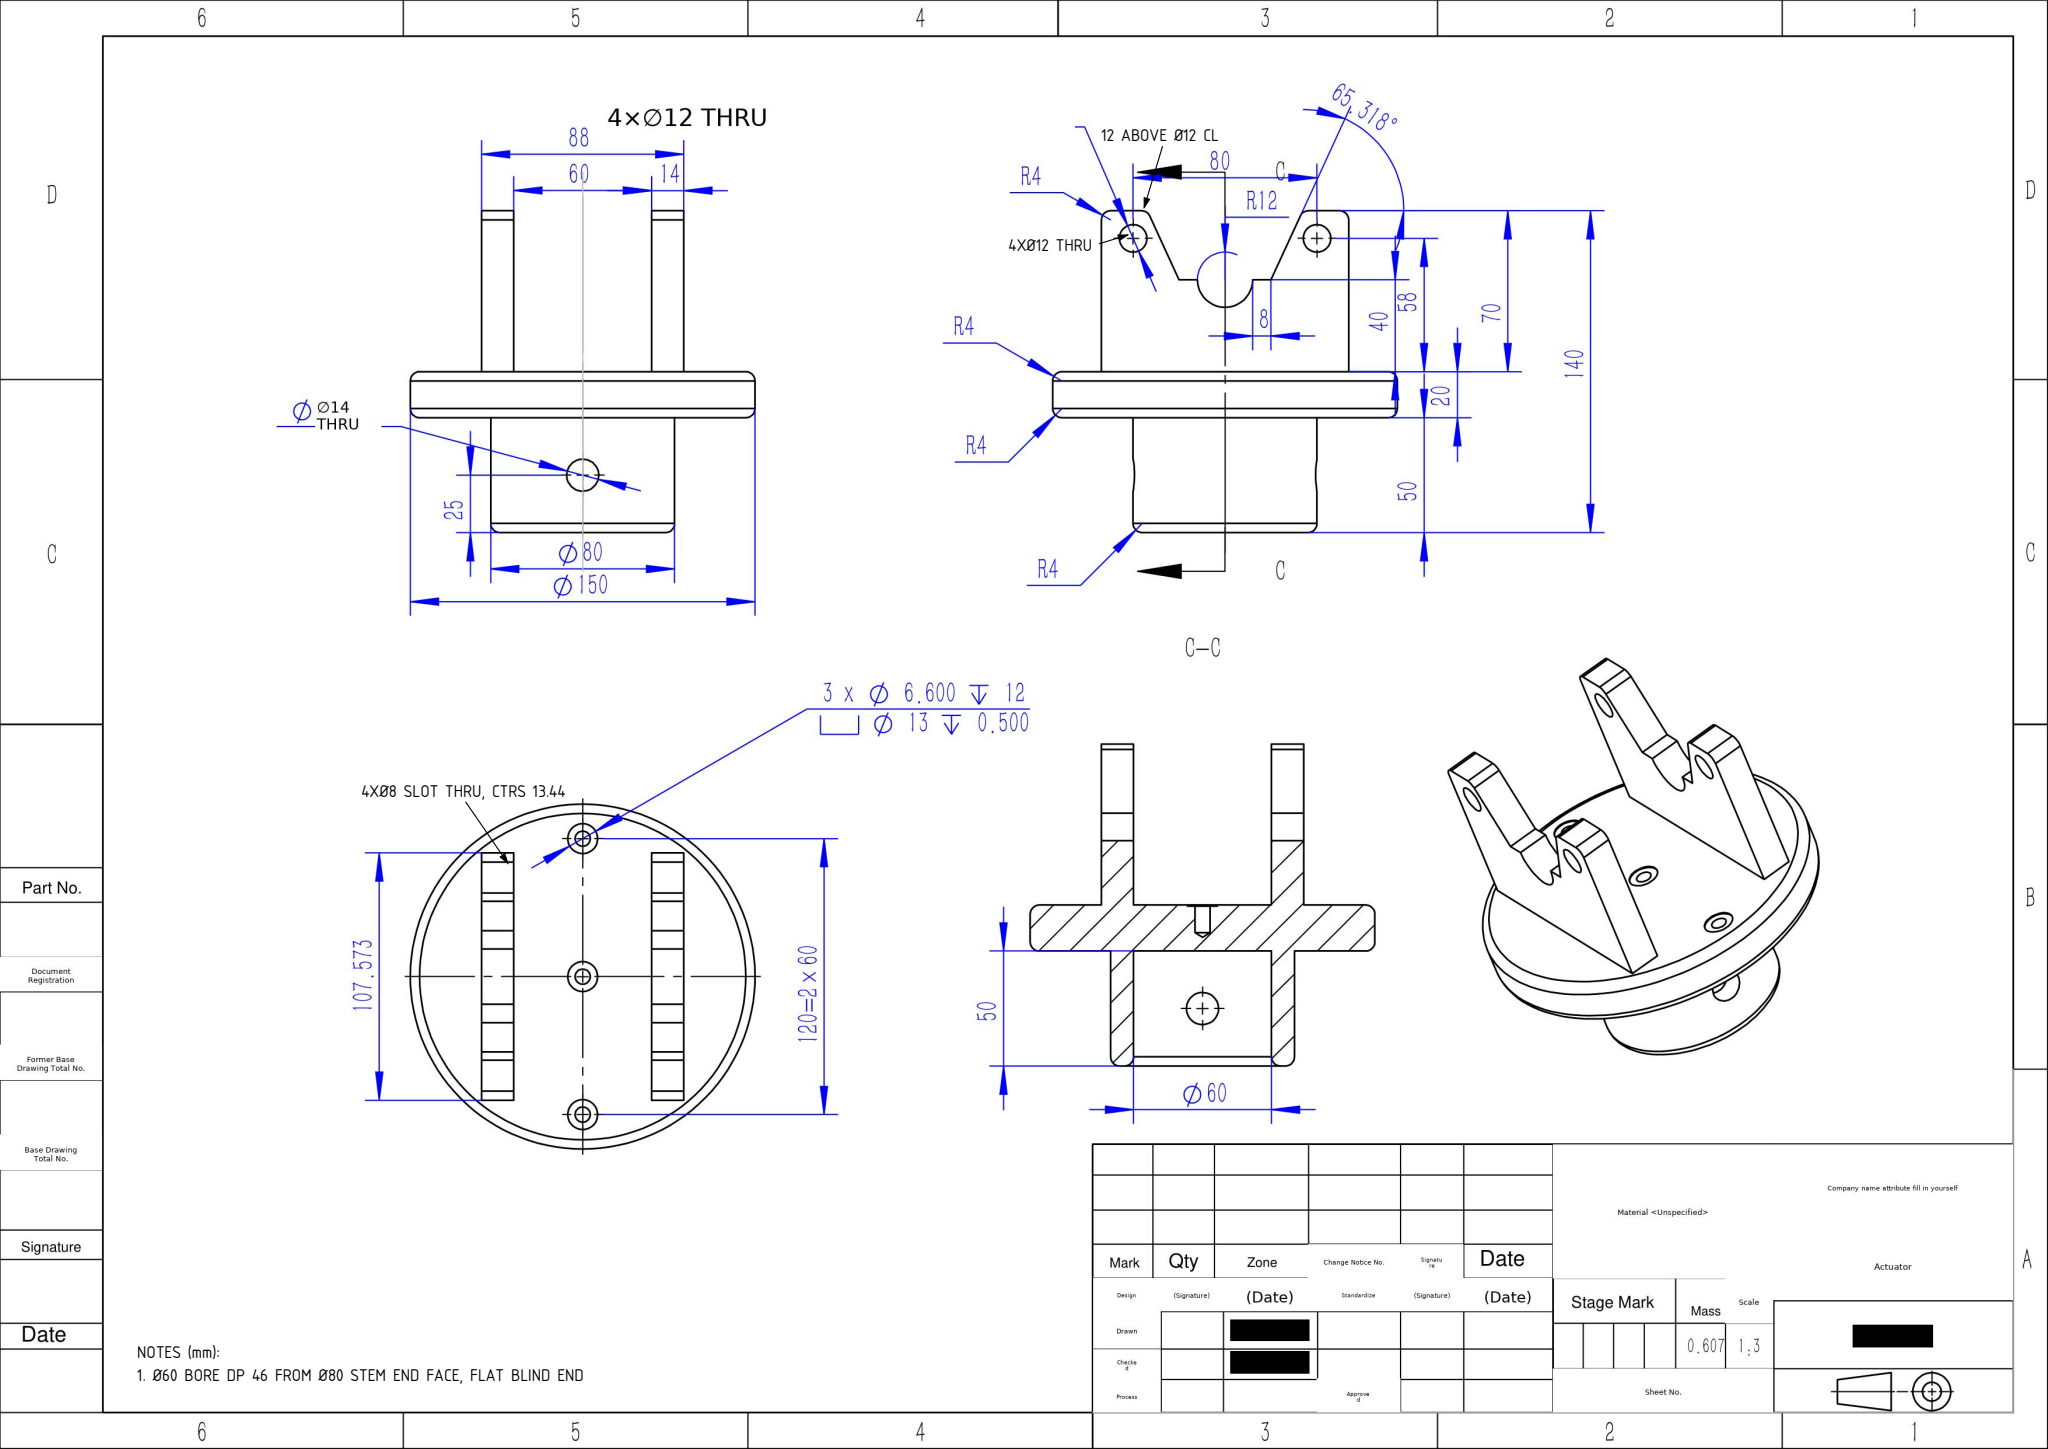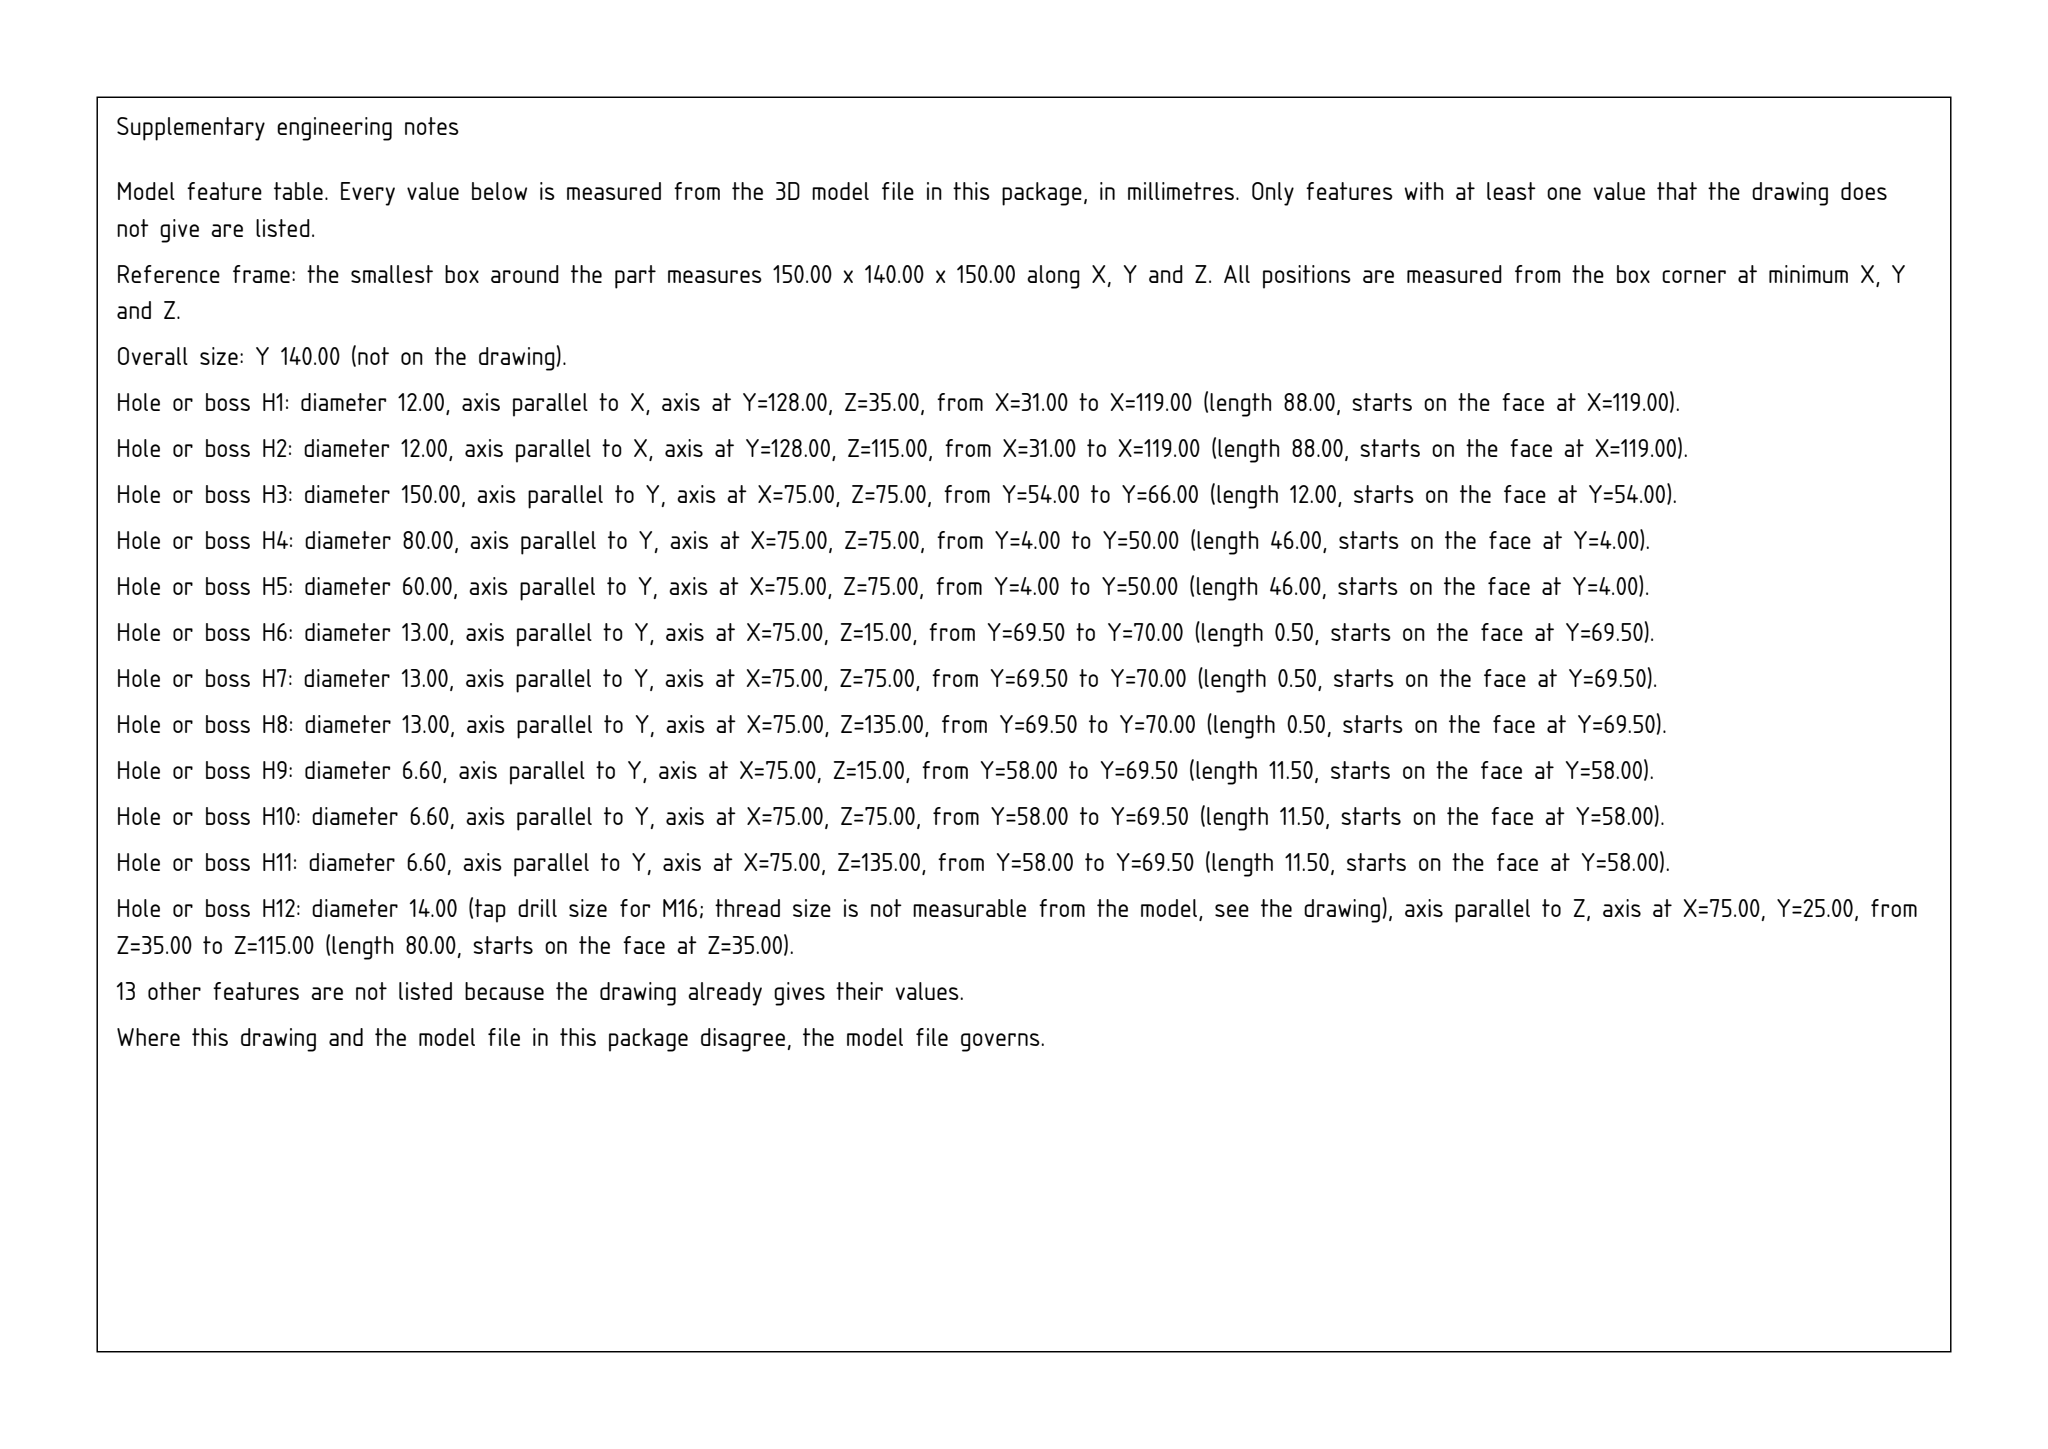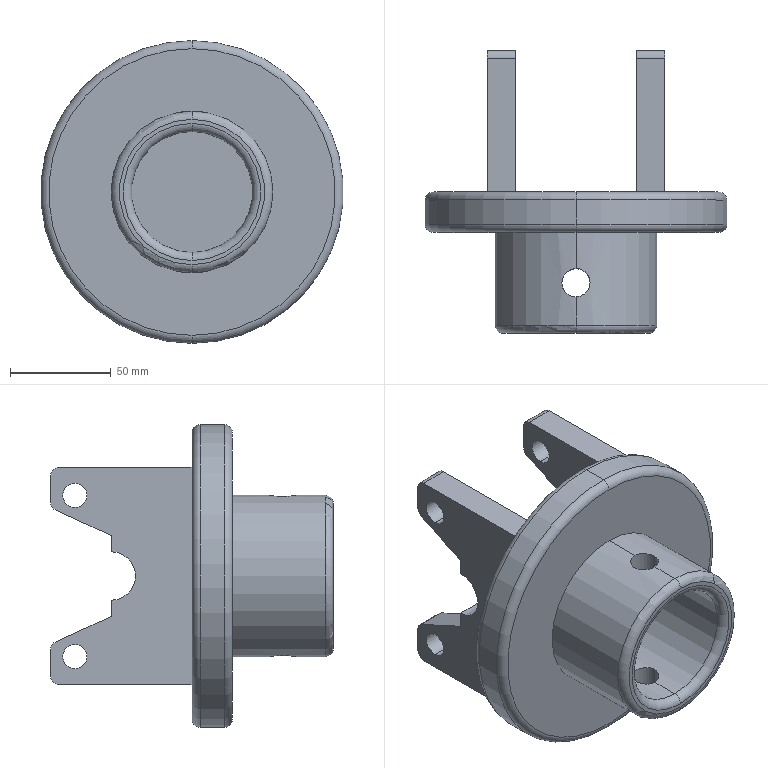Part | SolidWorks | mm | 1 solid | 81 faces | box 150 x 140 x 150 mm | volume 606876 mm3 | cylinder 40 | plane 27 | torus 8 | cone 6 | commonest cylinder face diameters 12 x8 8 x8 13 x6 6.6 x6 14 x4 150 x2 60 x2 80 x2
Drawing notes:
Ø60 BORE DP 46 FROM Ø80 STEM END FACE, FLAT BLIND END | from the solid: Ø60 y-axis cyl at [81.18,81.18] len 46; starts at stem end y=0, ends y=50, 4 below flange underside
4×Ø12 THRU AXES PERP FLANGE AXIS, 80 APART SYM ABT CL, CL 58 ABV FLANGE TOP | from the solid: Ø12 x-axis cyls at y=128, z=41.18 & 121.18; flange axis z=81.18 (±40); flange top plane y=70 → 128-70=58
PRONG TIP END FACE 12 ABV Ø12 CL; PRONG OUTR FACE 13.79 FROM Ø12 CL | from the solid: tip end face y=140 vs Ø12 axis y=128 → 12; Ø12 at z=41.18 vs prong outer face z=27.39 → 13.79
4×Ø8 THRU SLOT: CTRS 13.44 APART, 4 & 17.44 FROM PRONG OUTR FACE, CL 66 ABV FLANGE TOP | from the solid: Ø8 x-axis cyls y=136, z=31.39 & 44.83 (and 117.53 & 130.97), len 14 = prong thk; outer faces z=27.39/134.97; 136-70=66
build123d program:
from build123d import *

# Parameters (mm, degrees)
SKETCH1_R                                           = 40
SKETCH1_R_2                                         = 30
BOSS_EXTRUDE1_DEPTH                                 = 50
SKETCH2_R                                           = 75
BOSS_EXTRUDE2_DEPTH                                 = 20
BOSS_EXTRUDE3_START                                 = 30
BOSS_EXTRUDE3_DEPTH                                 = 14
CUT_EXTRUDE1_REACH                                  = 200.459
SKETCH5_R                                           = 6
CUT_EXTRUDE2_REACH                                  = 200.459
FILLET1_R                                           = 4
CYLINDRICAL_COUNTERSUNK_HOLE_FOR_M6_HEX_D           = 6.6
CYLINDRICAL_COUNTERSUNK_HOLE_FOR_M6_HEX_DEPTH       = 12
CYLINDRICAL_COUNTERSUNK_HOLE_FOR_M6_HEX_CBORE_D     = 13
CYLINDRICAL_COUNTERSUNK_HOLE_FOR_M6_HEX_CBORE_DEPTH = 0.5
CYLINDRICAL_COUNTERSUNK_HOLE_FOR_M6_HEX_TIP         = 1.983
FILLET2_R                                           = 4
CUT_EXTRUDE3_DEPTH                                  = 176.642
CUT_EXTRUDE3_DEPTH_BACK                             = 176.642
SKETCH10_R                                          = 7


with BuildPart() as part:
    # Sketch1 → Boss-Extrude1 (new body)
    with BuildSketch(Plane(origin=(0, 0, 0), x_dir=(1, 0, 0), z_dir=(0, 1, 0))):
        with Locations(Location((0, 0, 0), (0, 0, 270))):
            Circle(SKETCH1_R)
        with Locations(Location((0, 0, 0), (0, 0, 270))):
            Circle(SKETCH1_R_2, mode=Mode.SUBTRACT)
    extrude(amount=BOSS_EXTRUDE1_DEPTH)

    # Sketch2 → Boss-Extrude2 (add)
    with BuildSketch(Plane(origin=(0, 50, 0), x_dir=(1, 0, 0), z_dir=(0, 1, 0))):
        with Locations(Location((0, 0, 0), (0, 0, 270))):
            Circle(SKETCH2_R)
    extrude(amount=BOSS_EXTRUDE2_DEPTH)

    # Sketch4 → Boss-Extrude3 (add)
    with BuildSketch(Plane(origin=(0, 0, 0), x_dir=(0, 0, -1), z_dir=(1, 0, 0)).offset(BOSS_EXTRUDE3_START)):
        Polygon((-53.787, 140), (-53.787, 70), (53.787, 70), (53.787, 140), (33.787, 140), (20, 110), (-20, 110), (-33.787, 140), align=None)
    boss_extrude3 = extrude(amount=BOSS_EXTRUDE3_DEPTH)

    # Sketch5 → Cut-Extrude1 (cut, up to next)
    with BuildSketch(Plane(origin=(44, 0, 0), x_dir=(0, 0, -1), z_dir=(1, 0, 0)), mode=Mode.PRIVATE) as cut_extrude1_sk1:
        with Locations((-40, 128)):
            Circle(SKETCH5_R)
    cut_extrude1_tool1 = extrude(cut_extrude1_sk1.sketch, amount=-CUT_EXTRUDE1_REACH, mode=Mode.PRIVATE) & part.part
    # Sketch5 → Cut-Extrude1 (cut, up to next)
    with BuildSketch(Plane(origin=(44, 0, 0), x_dir=(0, 0, -1), z_dir=(1, 0, 0)), mode=Mode.PRIVATE) as cut_extrude1_sk2:
        with Locations((40, 128)):
            Circle(SKETCH5_R)
    cut_extrude1_tool2 = extrude(cut_extrude1_sk2.sketch, amount=-CUT_EXTRUDE1_REACH, mode=Mode.PRIVATE) & part.part
    cut_extrude1_1 = cut_extrude1_tool1.solids().sort_by_distance((44, 128, 40))[0]
    add(cut_extrude1_1, mode=Mode.SUBTRACT)
    cut_extrude1_2 = cut_extrude1_tool2.solids().sort_by_distance((44, 128, -40))[0]
    add(cut_extrude1_2, mode=Mode.SUBTRACT)
    cut_extrude1 = cut_extrude1_1 + cut_extrude1_2  # Cut-Extrude1 as one shape, for the pattern or mirror that repeats it

    # Sketch6 → Cut-Extrude2 (cut, up to next)
    with BuildSketch(Plane(origin=(44, 0, 0), x_dir=(0, 0, -1), z_dir=(1, 0, 0)), mode=Mode.PRIVATE) as cut_extrude2_sk1:
        with BuildLine():
            Line((-12, 110), (12, 110))
            ThreePointArc((12, 110), (0, 98), (-12, 110))
        make_face()
    cut_extrude2_tool1 = extrude(cut_extrude2_sk1.sketch, amount=-CUT_EXTRUDE2_REACH, mode=Mode.PRIVATE) & part.part
    cut_extrude2 = cut_extrude2_tool1.solids().sort_by_distance((44, 104.907, 0))[0]
    add(cut_extrude2, mode=Mode.SUBTRACT)

    # Mirror1: Boss-Extrude3, Cut-Extrude1, Cut-Extrude2 across plane
    add(boss_extrude3.mirror(Plane(origin=(0, 0, 0), x_dir=(0, 0, 1), z_dir=(1, 0, 0))))
    add(cut_extrude1.mirror(Plane(origin=(0, 0, 0), x_dir=(0, 0, 1), z_dir=(1, 0, 0))), mode=Mode.SUBTRACT)
    add(cut_extrude2.mirror(Plane(origin=(0, 0, 0), x_dir=(0, 0, 1), z_dir=(1, 0, 0))), mode=Mode.SUBTRACT)

    # Fillet1
    fillet1_edges = [part.edges().sort_by_distance(p)[0] for p in [
        (37, 140, 33.787),
        (37, 140, 53.787),
        (37, 140, -53.787),
        (37, 140, -33.787),
        (-37, 140, 53.787),
        (-37, 140, 33.787),
        (-37, 140, -33.787),
        (-37, 140, -53.787),
    ]]
    fillet(fillet1_edges, radius=FILLET1_R)

    # Cylindrical Countersunk Hole for M6 Hex
    with Locations(Plane(origin=(0, 70, 0), x_dir=(1, 0, 0), z_dir=(0, 1, 0))):
        with Locations((0, 60), (0, 0), (0, -60)):
            CounterBoreHole(CYLINDRICAL_COUNTERSUNK_HOLE_FOR_M6_HEX_D / 2, CYLINDRICAL_COUNTERSUNK_HOLE_FOR_M6_HEX_CBORE_D / 2, CYLINDRICAL_COUNTERSUNK_HOLE_FOR_M6_HEX_CBORE_DEPTH, depth=CYLINDRICAL_COUNTERSUNK_HOLE_FOR_M6_HEX_DEPTH)
            with Locations((0, 0, -(CYLINDRICAL_COUNTERSUNK_HOLE_FOR_M6_HEX_DEPTH + CYLINDRICAL_COUNTERSUNK_HOLE_FOR_M6_HEX_TIP / 2))):  # 118° drill point
                Cone(0, CYLINDRICAL_COUNTERSUNK_HOLE_FOR_M6_HEX_D / 2, CYLINDRICAL_COUNTERSUNK_HOLE_FOR_M6_HEX_TIP, mode=Mode.SUBTRACT)

    # Fillet2
    fillet2_edges = [part.edges().sort_by_distance(p)[0] for p in [
        (0, 50, -75),
        (0, 70, -75),
        (0, 0, -40),
        (0, 0, -30),
    ]]
    fillet(fillet2_edges, radius=FILLET2_R)

    # Sketch10 → Cut-Extrude3 (cut, two sides: drawn at the far end of the back side and taken through both)
    with BuildSketch(Plane.XY.offset(-CUT_EXTRUDE3_DEPTH_BACK)):
        with Locations((0, 25)):
            Circle(SKETCH10_R)
    extrude(amount=CUT_EXTRUDE3_DEPTH + CUT_EXTRUDE3_DEPTH_BACK, mode=Mode.SUBTRACT)


solid = part.part